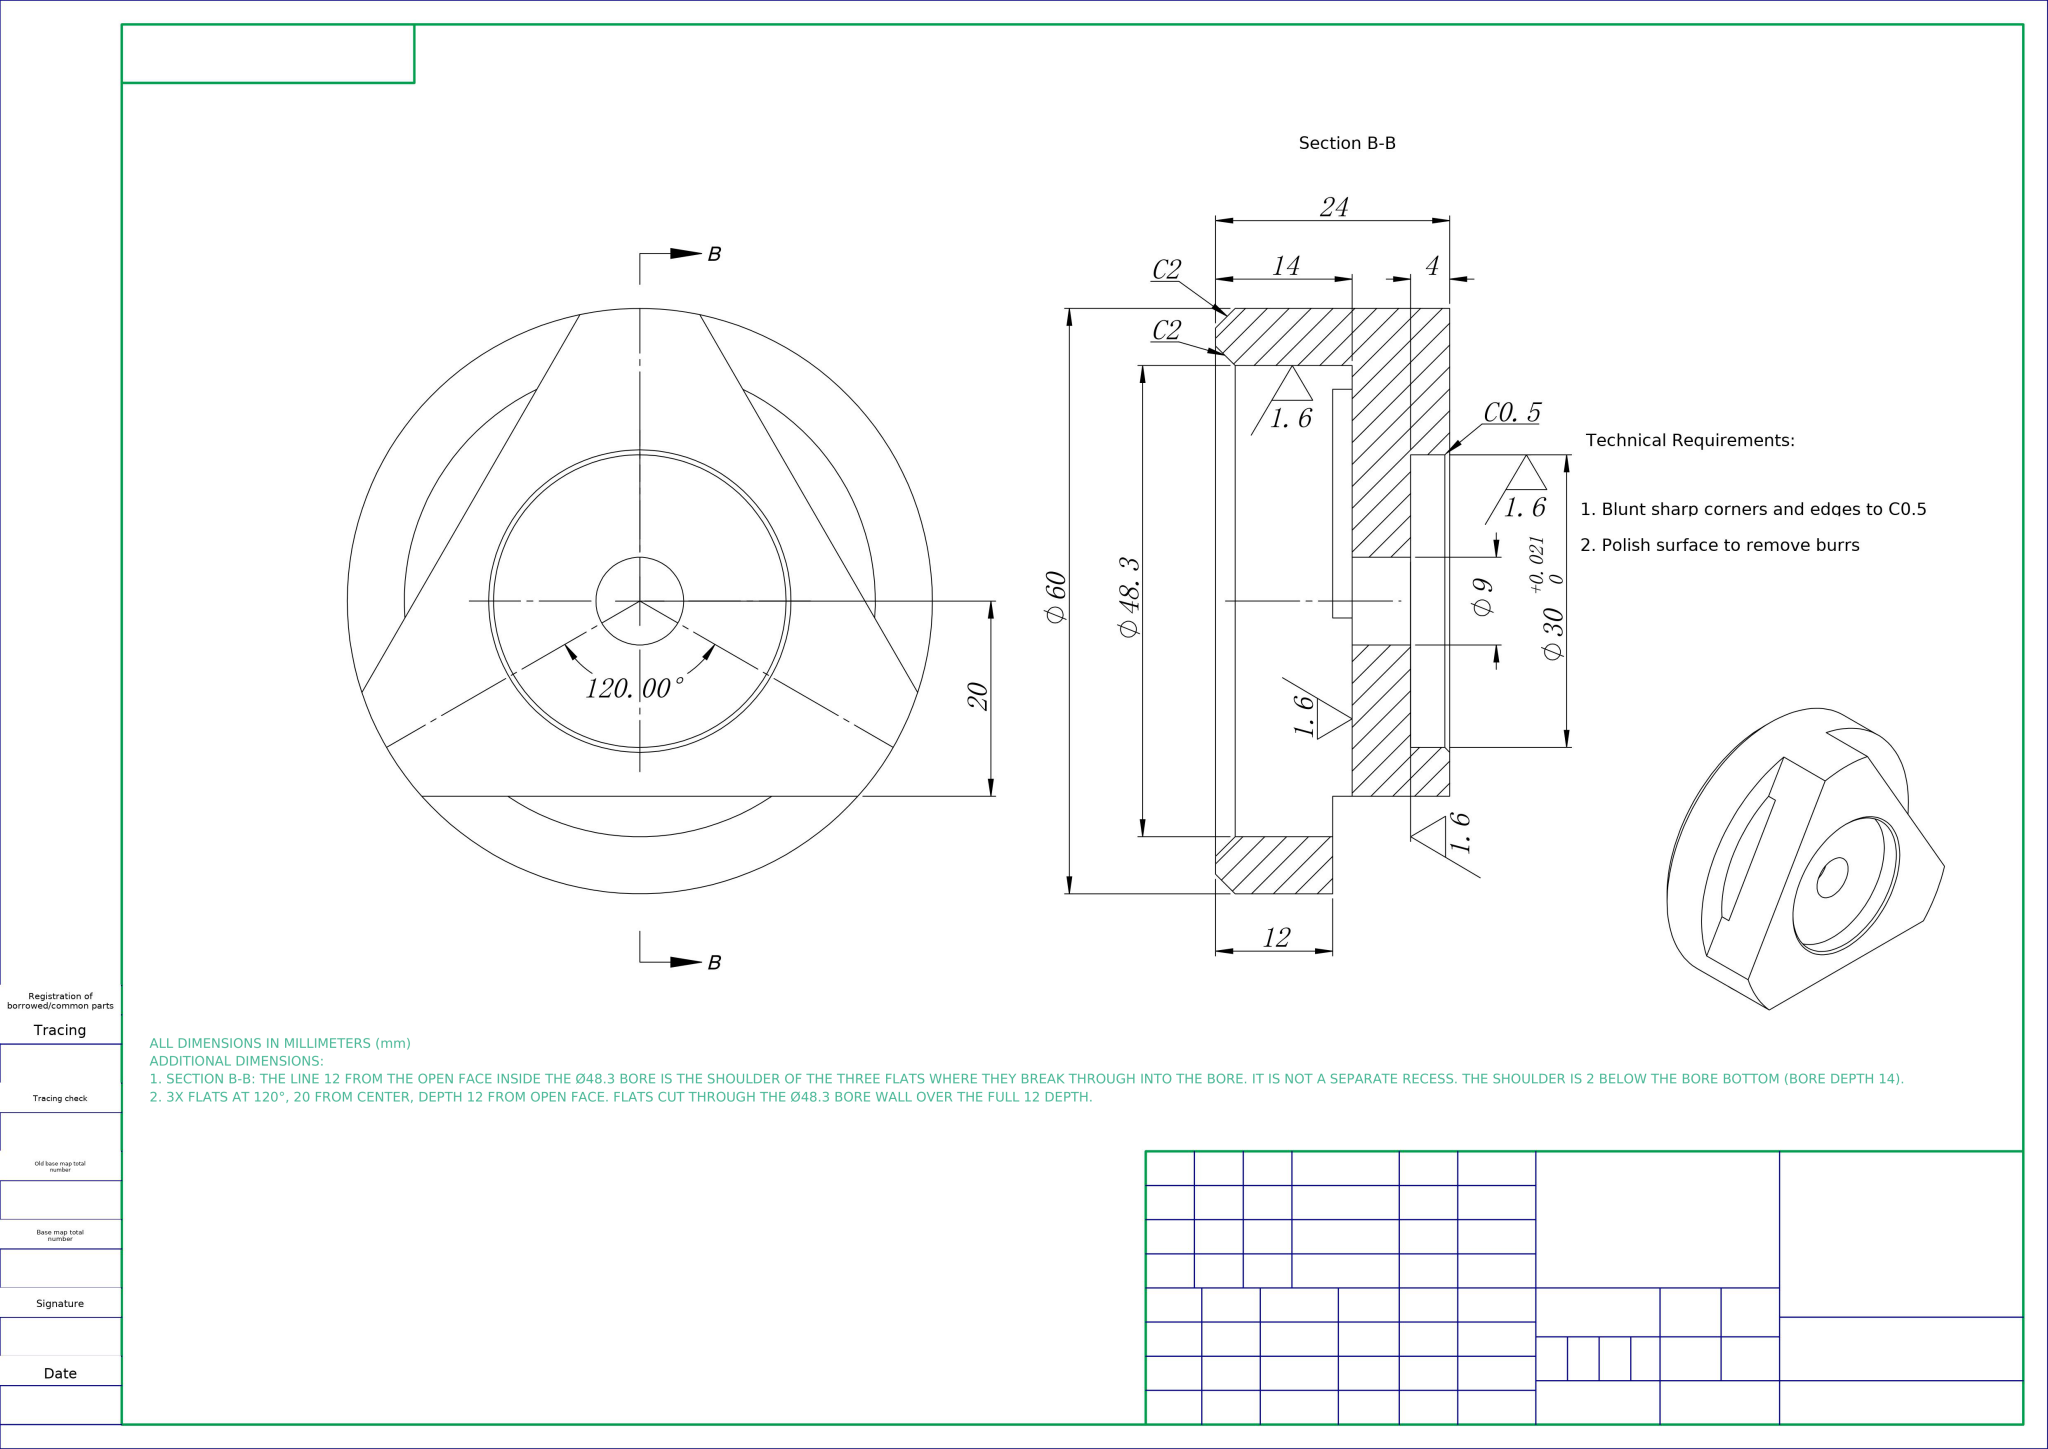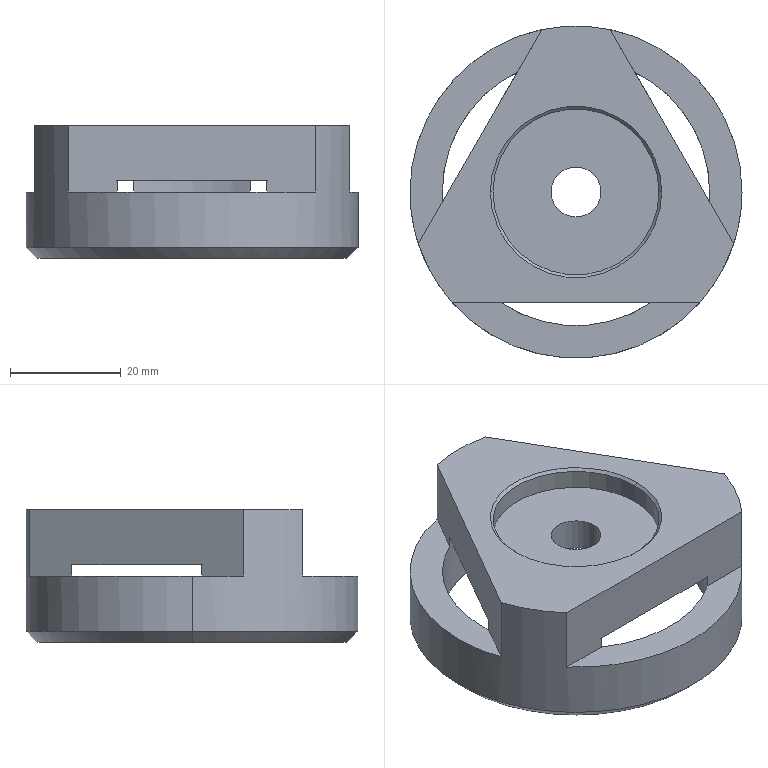Part | NX | mm | 1 solid | 24 faces | box 60 x 60 x 24 mm | volume 27612 mm3 | plane 10 | cylinder 8 | cone 6 | commonest cylinder face diameters 30 x2 48.3 x2 60 x2 9 x2
STEP:
#1=COLOUR_RGB('',0.,1.,1.);
#2=FILL_AREA_STYLE_COLOUR('',#1);
#3=FILL_AREA_STYLE('',(#2));
#4=SURFACE_STYLE_FILL_AREA(#3);
#5=SURFACE_SIDE_STYLE('',(#4));
#6=SURFACE_STYLE_USAGE(.BOTH.,#5);
#7=PRESENTATION_STYLE_ASSIGNMENT((#6));
#8=CARTESIAN_POINT('',(-15.,0.,23.5));
#9=VERTEX_POINT('',#8);
#10=CARTESIAN_POINT('',(15.,0.,23.5));
#11=VERTEX_POINT('',#10);
#12=CARTESIAN_POINT('',(0.,0.,23.5));
#13=DIRECTION('',(0.,0.,1.));
#14=DIRECTION('',(1.,0.,0.));
#15=AXIS2_PLACEMENT_3D('',#12,#13,#14);
#16=CIRCLE('',#15,15.);
#17=EDGE_CURVE('',#9,#11,#16,.T.);
#18=ORIENTED_EDGE('',*,*,#17,.F.);
#19=CARTESIAN_POINT('',(-15.5,0.,24.));
#20=VERTEX_POINT('',#19);
#21=CARTESIAN_POINT('',(-15.,0.,23.5));
#22=DIRECTION('',(-0.7071,0.,0.7071));
#23=VECTOR('',#22,1000.);
#24=LINE('',#21,#23);
#25=EDGE_CURVE('',#9,#20,#24,.T.);
#26=ORIENTED_EDGE('',*,*,#25,.T.);
#27=CARTESIAN_POINT('',(15.5,0.,24.));
#28=VERTEX_POINT('',#27);
#29=CARTESIAN_POINT('',(0.,0.,24.));
#30=DIRECTION('',(0.,0.,-1.));
#31=DIRECTION('',(1.,0.,0.));
#32=AXIS2_PLACEMENT_3D('',#29,#30,#31);
#33=CIRCLE('',#32,15.5);
#34=EDGE_CURVE('',#28,#20,#33,.T.);
#35=ORIENTED_EDGE('',*,*,#34,.F.);
#36=CARTESIAN_POINT('',(15.,0.,23.5));
#37=DIRECTION('',(0.7071,0.,0.7071));
#38=VECTOR('',#37,1000.);
#39=LINE('',#36,#38);
#40=EDGE_CURVE('',#11,#28,#39,.T.);
#41=ORIENTED_EDGE('',*,*,#40,.F.);
#42=EDGE_LOOP('',(#18,#26,#35,#41));
#43=FACE_OUTER_BOUND('',#42,.T.);
#44=CARTESIAN_POINT('',(0.,0.,23.5));
#45=DIRECTION('',(0.,0.,1.));
#46=DIRECTION('',(1.,0.,0.));
#47=AXIS2_PLACEMENT_3D('',#44,#45,#46);
#48=CONICAL_SURFACE('',#47,15.,0.7854);
#49=ADVANCED_FACE('',(#43),#48,.F.);
#50=CARTESIAN_POINT('',(-15.,0.,20.));
#51=VERTEX_POINT('',#50);
#52=CARTESIAN_POINT('',(15.,0.,20.));
#53=VERTEX_POINT('',#52);
#54=CARTESIAN_POINT('',(0.,0.,20.));
#55=DIRECTION('',(0.,0.,1.));
#56=DIRECTION('',(1.,0.,0.));
#57=AXIS2_PLACEMENT_3D('',#54,#55,#56);
#58=CIRCLE('',#57,15.);
#59=EDGE_CURVE('',#51,#53,#58,.T.);
#60=ORIENTED_EDGE('',*,*,#59,.F.);
#61=CARTESIAN_POINT('',(-15.,0.,20.));
#62=DIRECTION('',(0.,0.,1.));
#63=VECTOR('',#62,1000.);
#64=LINE('',#61,#63);
#65=EDGE_CURVE('',#51,#9,#64,.T.);
#66=ORIENTED_EDGE('',*,*,#65,.T.);
#67=ORIENTED_EDGE('',*,*,#17,.T.);
#68=CARTESIAN_POINT('',(15.,0.,20.));
#69=DIRECTION('',(0.,0.,1.));
#70=VECTOR('',#69,1000.);
#71=LINE('',#68,#70);
#72=EDGE_CURVE('',#53,#11,#71,.T.);
#73=ORIENTED_EDGE('',*,*,#72,.F.);
#74=EDGE_LOOP('',(#60,#66,#67,#73));
#75=FACE_OUTER_BOUND('',#74,.T.);
#76=CARTESIAN_POINT('',(0.,0.,20.));
#77=DIRECTION('',(0.,0.,1.));
#78=DIRECTION('',(1.,0.,0.));
#79=AXIS2_PLACEMENT_3D('',#76,#77,#78);
#80=CYLINDRICAL_SURFACE('',#79,15.);
#81=ADVANCED_FACE('',(#75),#80,.F.);
#82=CARTESIAN_POINT('',(24.15,0.,2.));
#83=VERTEX_POINT('',#82);
#84=CARTESIAN_POINT('',(-24.15,0.,2.));
#85=VERTEX_POINT('',#84);
#86=CARTESIAN_POINT('',(0.,0.,2.));
#87=DIRECTION('',(0.,0.,-1.));
#88=DIRECTION('',(1.,0.,0.));
#89=AXIS2_PLACEMENT_3D('',#86,#87,#88);
#90=CIRCLE('',#89,24.15);
#91=EDGE_CURVE('',#83,#85,#90,.T.);
#92=ORIENTED_EDGE('',*,*,#91,.F.);
#93=CARTESIAN_POINT('',(26.15,0.,0.));
#94=VERTEX_POINT('',#93);
#95=CARTESIAN_POINT('',(26.15,0.,0.));
#96=DIRECTION('',(0.7071,0.,-0.7071));
#97=VECTOR('',#96,1000.);
#98=LINE('',#95,#97);
#99=EDGE_CURVE('',#83,#94,#98,.T.);
#100=ORIENTED_EDGE('',*,*,#99,.T.);
#101=CARTESIAN_POINT('',(-26.15,0.,0.));
#102=VERTEX_POINT('',#101);
#103=CARTESIAN_POINT('',(0.,0.,0.));
#104=DIRECTION('',(0.,0.,1.));
#105=DIRECTION('',(1.,0.,0.));
#106=AXIS2_PLACEMENT_3D('',#103,#104,#105);
#107=CIRCLE('',#106,26.15);
#108=EDGE_CURVE('',#102,#94,#107,.T.);
#109=ORIENTED_EDGE('',*,*,#108,.F.);
#110=CARTESIAN_POINT('',(-26.15,0.,0.));
#111=DIRECTION('',(-0.7071,0.,-0.7071));
#112=VECTOR('',#111,1000.);
#113=LINE('',#110,#112);
#114=EDGE_CURVE('',#85,#102,#113,.T.);
#115=ORIENTED_EDGE('',*,*,#114,.F.);
#116=EDGE_LOOP('',(#92,#100,#109,#115));
#117=FACE_OUTER_BOUND('',#116,.T.);
#118=CARTESIAN_POINT('',(0.,0.,0.));
#119=DIRECTION('',(0.,0.,-1.));
#120=DIRECTION('',(-1.,0.,0.));
#121=AXIS2_PLACEMENT_3D('',#118,#119,#120);
#122=CONICAL_SURFACE('',#121,26.15,0.7854);
#123=ADVANCED_FACE('',(#117),#122,.F.);
#124=CARTESIAN_POINT('',(-28.,0.,0.));
#125=VERTEX_POINT('',#124);
#126=CARTESIAN_POINT('',(28.,0.,0.));
#127=VERTEX_POINT('',#126);
#128=CARTESIAN_POINT('',(0.,0.,0.));
#129=DIRECTION('',(0.,0.,-1.));
#130=DIRECTION('',(1.,0.,0.));
#131=AXIS2_PLACEMENT_3D('',#128,#129,#130);
#132=CIRCLE('',#131,28.);
#133=EDGE_CURVE('',#125,#127,#132,.T.);
#134=ORIENTED_EDGE('',*,*,#133,.F.);
#135=CARTESIAN_POINT('',(-30.,0.,2.));
#136=VERTEX_POINT('',#135);
#137=CARTESIAN_POINT('',(-30.,0.,2.));
#138=DIRECTION('',(-0.7071,0.,0.7071));
#139=VECTOR('',#138,1000.);
#140=LINE('',#137,#139);
#141=EDGE_CURVE('',#125,#136,#140,.T.);
#142=ORIENTED_EDGE('',*,*,#141,.T.);
#143=CARTESIAN_POINT('',(30.,0.,2.));
#144=VERTEX_POINT('',#143);
#145=CARTESIAN_POINT('',(0.,0.,2.));
#146=DIRECTION('',(0.,0.,1.));
#147=DIRECTION('',(1.,0.,0.));
#148=AXIS2_PLACEMENT_3D('',#145,#146,#147);
#149=CIRCLE('',#148,30.);
#150=EDGE_CURVE('',#144,#136,#149,.T.);
#151=ORIENTED_EDGE('',*,*,#150,.F.);
#152=CARTESIAN_POINT('',(30.,0.,2.));
#153=DIRECTION('',(0.7071,0.,0.7071));
#154=VECTOR('',#153,1000.);
#155=LINE('',#152,#154);
#156=EDGE_CURVE('',#127,#144,#155,.T.);
#157=ORIENTED_EDGE('',*,*,#156,.F.);
#158=EDGE_LOOP('',(#134,#142,#151,#157));
#159=FACE_OUTER_BOUND('',#158,.T.);
#160=CARTESIAN_POINT('',(0.,0.,2.));
#161=DIRECTION('',(0.,0.,1.));
#162=DIRECTION('',(1.,0.,0.));
#163=AXIS2_PLACEMENT_3D('',#160,#161,#162);
#164=CONICAL_SURFACE('',#163,30.,0.7854);
#165=ADVANCED_FACE('',(#159),#164,.T.);
#166=CARTESIAN_POINT('',(24.088,-1.722,12.));
#167=VERTEX_POINT('',#166);
#168=CARTESIAN_POINT('',(24.15,0.,12.));
#169=VERTEX_POINT('',#168);
#170=CARTESIAN_POINT('',(0.,0.,12.));
#171=DIRECTION('',(0.,0.,1.));
#172=DIRECTION('',(1.,0.,0.));
#173=AXIS2_PLACEMENT_3D('',#170,#171,#172);
#174=CIRCLE('',#173,24.15);
#175=EDGE_CURVE('',#167,#169,#174,.T.);
#176=ORIENTED_EDGE('',*,*,#175,.T.);
#177=CARTESIAN_POINT('',(24.15,0.,14.));
#178=DIRECTION('',(0.,0.,-1.));
#179=VECTOR('',#178,1000.);
#180=LINE('',#177,#179);
#181=EDGE_CURVE('',#169,#83,#180,.T.);
#182=ORIENTED_EDGE('',*,*,#181,.T.);
#183=ORIENTED_EDGE('',*,*,#91,.T.);
#184=CARTESIAN_POINT('',(-24.15,0.,12.));
#185=VERTEX_POINT('',#184);
#186=CARTESIAN_POINT('',(-24.15,0.,14.));
#187=DIRECTION('',(0.,0.,-1.));
#188=VECTOR('',#187,1000.);
#189=LINE('',#186,#188);
#190=EDGE_CURVE('',#185,#85,#189,.T.);
#191=ORIENTED_EDGE('',*,*,#190,.F.);
#192=CARTESIAN_POINT('',(-24.088,-1.722,12.));
#193=VERTEX_POINT('',#192);
#194=CARTESIAN_POINT('',(0.,0.,12.));
#195=DIRECTION('',(0.,0.,1.));
#196=DIRECTION('',(1.,0.,0.));
#197=AXIS2_PLACEMENT_3D('',#194,#195,#196);
#198=CIRCLE('',#197,24.15);
#199=EDGE_CURVE('',#185,#193,#198,.T.);
#200=ORIENTED_EDGE('',*,*,#199,.T.);
#201=CARTESIAN_POINT('',(-24.088,-1.722,14.));
#202=VERTEX_POINT('',#201);
#203=CARTESIAN_POINT('',(-24.088,-1.722,14.));
#204=DIRECTION('',(0.,0.,-1.));
#205=VECTOR('',#204,1000.);
#206=LINE('',#203,#205);
#207=EDGE_CURVE('',#202,#193,#206,.T.);
#208=ORIENTED_EDGE('',*,*,#207,.F.);
#209=CARTESIAN_POINT('',(-13.536,-20.,14.));
#210=VERTEX_POINT('',#209);
#211=CARTESIAN_POINT('',(0.,0.,14.));
#212=DIRECTION('',(0.,0.,1.));
#213=DIRECTION('',(1.,0.,0.));
#214=AXIS2_PLACEMENT_3D('',#211,#212,#213);
#215=CIRCLE('',#214,24.15);
#216=EDGE_CURVE('',#202,#210,#215,.T.);
#217=ORIENTED_EDGE('',*,*,#216,.T.);
#218=CARTESIAN_POINT('',(-13.536,-20.,12.));
#219=VERTEX_POINT('',#218);
#220=CARTESIAN_POINT('',(-13.536,-20.,14.));
#221=DIRECTION('',(0.,0.,1.));
#222=VECTOR('',#221,1000.);
#223=LINE('',#220,#222);
#224=EDGE_CURVE('',#219,#210,#223,.T.);
#225=ORIENTED_EDGE('',*,*,#224,.F.);
#226=CARTESIAN_POINT('',(13.536,-20.,12.));
#227=VERTEX_POINT('',#226);
#228=CARTESIAN_POINT('',(0.,0.,12.));
#229=DIRECTION('',(0.,0.,1.));
#230=DIRECTION('',(1.,0.,0.));
#231=AXIS2_PLACEMENT_3D('',#228,#229,#230);
#232=CIRCLE('',#231,24.15);
#233=EDGE_CURVE('',#219,#227,#232,.T.);
#234=ORIENTED_EDGE('',*,*,#233,.T.);
#235=CARTESIAN_POINT('',(13.536,-20.,14.));
#236=VERTEX_POINT('',#235);
#237=CARTESIAN_POINT('',(13.536,-20.,14.));
#238=DIRECTION('',(0.,0.,-1.));
#239=VECTOR('',#238,1000.);
#240=LINE('',#237,#239);
#241=EDGE_CURVE('',#236,#227,#240,.T.);
#242=ORIENTED_EDGE('',*,*,#241,.F.);
#243=CARTESIAN_POINT('',(24.088,-1.722,14.));
#244=VERTEX_POINT('',#243);
#245=CARTESIAN_POINT('',(0.,0.,14.));
#246=DIRECTION('',(0.,0.,1.));
#247=DIRECTION('',(1.,0.,0.));
#248=AXIS2_PLACEMENT_3D('',#245,#246,#247);
#249=CIRCLE('',#248,24.15);
#250=EDGE_CURVE('',#236,#244,#249,.T.);
#251=ORIENTED_EDGE('',*,*,#250,.T.);
#252=CARTESIAN_POINT('',(24.088,-1.722,14.));
#253=DIRECTION('',(0.,0.,1.));
#254=VECTOR('',#253,1000.);
#255=LINE('',#252,#254);
#256=EDGE_CURVE('',#167,#244,#255,.T.);
#257=ORIENTED_EDGE('',*,*,#256,.F.);
#258=EDGE_LOOP('',(#176,#182,#183,#191,#200,#208,#217,#225,#234,#242,#251,#257));
#259=FACE_OUTER_BOUND('',#258,.T.);
#260=CARTESIAN_POINT('',(0.,0.,14.));
#261=DIRECTION('',(0.,0.,-1.));
#262=DIRECTION('',(-1.,0.,0.));
#263=AXIS2_PLACEMENT_3D('',#260,#261,#262);
#264=CYLINDRICAL_SURFACE('',#263,24.15);
#265=ADVANCED_FACE('',(#259),#264,.F.);
#266=CARTESIAN_POINT('',(30.,0.,12.));
#267=VERTEX_POINT('',#266);
#268=CARTESIAN_POINT('',(6.14,29.365,12.));
#269=VERTEX_POINT('',#268);
#270=CARTESIAN_POINT('',(0.,0.,12.));
#271=DIRECTION('',(0.,0.,1.));
#272=DIRECTION('',(-0.5,-0.866,0.));
#273=AXIS2_PLACEMENT_3D('',#270,#271,#272);
#274=CIRCLE('',#273,30.);
#275=EDGE_CURVE('',#267,#269,#274,.T.);
#276=ORIENTED_EDGE('',*,*,#275,.F.);
#277=CARTESIAN_POINT('',(30.,0.,14.));
#278=DIRECTION('',(0.,0.,-1.));
#279=VECTOR('',#278,1000.);
#280=LINE('',#277,#279);
#281=EDGE_CURVE('',#267,#144,#280,.T.);
#282=ORIENTED_EDGE('',*,*,#281,.T.);
#283=ORIENTED_EDGE('',*,*,#150,.T.);
#284=CARTESIAN_POINT('',(-30.,0.,12.));
#285=VERTEX_POINT('',#284);
#286=CARTESIAN_POINT('',(-30.,0.,14.));
#287=DIRECTION('',(0.,0.,-1.));
#288=VECTOR('',#287,1000.);
#289=LINE('',#286,#288);
#290=EDGE_CURVE('',#285,#136,#289,.T.);
#291=ORIENTED_EDGE('',*,*,#290,.F.);
#292=CARTESIAN_POINT('',(-6.14,29.365,12.));
#293=VERTEX_POINT('',#292);
#294=CARTESIAN_POINT('',(0.,0.,12.));
#295=DIRECTION('',(0.,0.,1.));
#296=DIRECTION('',(1.,0.,0.));
#297=AXIS2_PLACEMENT_3D('',#294,#295,#296);
#298=CIRCLE('',#297,30.);
#299=EDGE_CURVE('',#293,#285,#298,.T.);
#300=ORIENTED_EDGE('',*,*,#299,.F.);
#301=CARTESIAN_POINT('',(-6.14,29.365,24.));
#302=VERTEX_POINT('',#301);
#303=CARTESIAN_POINT('',(-6.14,29.365,12.));
#304=DIRECTION('',(0.,0.,1.));
#305=VECTOR('',#304,1000.);
#306=LINE('',#303,#305);
#307=EDGE_CURVE('',#293,#302,#306,.T.);
#308=ORIENTED_EDGE('',*,*,#307,.T.);
#309=CARTESIAN_POINT('',(6.14,29.365,24.));
#310=VERTEX_POINT('',#309);
#311=CARTESIAN_POINT('',(0.,0.,24.));
#312=DIRECTION('',(0.,0.,1.));
#313=DIRECTION('',(1.,0.,0.));
#314=AXIS2_PLACEMENT_3D('',#311,#312,#313);
#315=CIRCLE('',#314,30.);
#316=EDGE_CURVE('',#310,#302,#315,.T.);
#317=ORIENTED_EDGE('',*,*,#316,.F.);
#318=CARTESIAN_POINT('',(6.14,29.365,12.));
#319=DIRECTION('',(0.,0.,1.));
#320=VECTOR('',#319,1000.);
#321=LINE('',#318,#320);
#322=EDGE_CURVE('',#269,#310,#321,.T.);
#323=ORIENTED_EDGE('',*,*,#322,.F.);
#324=EDGE_LOOP('',(#276,#282,#283,#291,#300,#308,#317,#323));
#325=FACE_OUTER_BOUND('',#324,.T.);
#326=CARTESIAN_POINT('',(0.,0.,14.));
#327=DIRECTION('',(0.,0.,-1.));
#328=DIRECTION('',(-1.,0.,0.));
#329=AXIS2_PLACEMENT_3D('',#326,#327,#328);
#330=CYLINDRICAL_SURFACE('',#329,30.);
#331=ADVANCED_FACE('',(#325),#330,.T.);
#332=CARTESIAN_POINT('',(4.5,0.,20.));
#333=VERTEX_POINT('',#332);
#334=CARTESIAN_POINT('',(-4.5,0.,20.));
#335=VERTEX_POINT('',#334);
#336=CARTESIAN_POINT('',(0.,0.,20.));
#337=DIRECTION('',(0.,0.,-1.));
#338=DIRECTION('',(1.,0.,0.));
#339=AXIS2_PLACEMENT_3D('',#336,#337,#338);
#340=CIRCLE('',#339,4.5);
#341=EDGE_CURVE('',#333,#335,#340,.T.);
#342=ORIENTED_EDGE('',*,*,#341,.F.);
#343=CARTESIAN_POINT('',(4.5,0.,14.));
#344=VERTEX_POINT('',#343);
#345=CARTESIAN_POINT('',(4.5,0.,14.));
#346=DIRECTION('',(0.,0.,-1.));
#347=VECTOR('',#346,1000.);
#348=LINE('',#345,#347);
#349=EDGE_CURVE('',#333,#344,#348,.T.);
#350=ORIENTED_EDGE('',*,*,#349,.T.);
#351=CARTESIAN_POINT('',(-4.5,0.,14.));
#352=VERTEX_POINT('',#351);
#353=CARTESIAN_POINT('',(0.,0.,14.));
#354=DIRECTION('',(0.,0.,-1.));
#355=DIRECTION('',(-1.,0.,0.));
#356=AXIS2_PLACEMENT_3D('',#353,#354,#355);
#357=CIRCLE('',#356,4.5);
#358=EDGE_CURVE('',#344,#352,#357,.T.);
#359=ORIENTED_EDGE('',*,*,#358,.T.);
#360=CARTESIAN_POINT('',(-4.5,0.,14.));
#361=DIRECTION('',(0.,0.,-1.));
#362=VECTOR('',#361,1000.);
#363=LINE('',#360,#362);
#364=EDGE_CURVE('',#335,#352,#363,.T.);
#365=ORIENTED_EDGE('',*,*,#364,.F.);
#366=EDGE_LOOP('',(#342,#350,#359,#365));
#367=FACE_OUTER_BOUND('',#366,.T.);
#368=CARTESIAN_POINT('',(0.,0.,14.));
#369=DIRECTION('',(0.,0.,-1.));
#370=DIRECTION('',(-1.,0.,0.));
#371=AXIS2_PLACEMENT_3D('',#368,#369,#370);
#372=CYLINDRICAL_SURFACE('',#371,4.5);
#373=ADVANCED_FACE('',(#367),#372,.F.);
#374=ORIENTED_EDGE('',*,*,#349,.F.);
#375=CARTESIAN_POINT('',(0.,0.,20.));
#376=DIRECTION('',(0.,0.,-1.));
#377=DIRECTION('',(1.,0.,0.));
#378=AXIS2_PLACEMENT_3D('',#375,#376,#377);
#379=CIRCLE('',#378,4.5);
#380=EDGE_CURVE('',#335,#333,#379,.T.);
#381=ORIENTED_EDGE('',*,*,#380,.F.);
#382=ORIENTED_EDGE('',*,*,#364,.T.);
#383=CARTESIAN_POINT('',(0.,0.,14.));
#384=DIRECTION('',(0.,0.,-1.));
#385=DIRECTION('',(-1.,0.,0.));
#386=AXIS2_PLACEMENT_3D('',#383,#384,#385);
#387=CIRCLE('',#386,4.5);
#388=EDGE_CURVE('',#352,#344,#387,.T.);
#389=ORIENTED_EDGE('',*,*,#388,.T.);
#390=EDGE_LOOP('',(#374,#381,#382,#389));
#391=FACE_OUTER_BOUND('',#390,.T.);
#392=CARTESIAN_POINT('',(0.,0.,14.));
#393=DIRECTION('',(0.,0.,-1.));
#394=DIRECTION('',(-1.,0.,0.));
#395=AXIS2_PLACEMENT_3D('',#392,#393,#394);
#396=CYLINDRICAL_SURFACE('',#395,4.5);
#397=ADVANCED_FACE('',(#391),#396,.F.);
#398=CARTESIAN_POINT('',(0.,0.,0.));
#399=DIRECTION('',(0.,0.,-1.));
#400=DIRECTION('',(1.,0.,0.));
#401=AXIS2_PLACEMENT_3D('',#398,#399,#400);
#402=CIRCLE('',#401,28.);
#403=EDGE_CURVE('',#127,#125,#402,.T.);
#404=ORIENTED_EDGE('',*,*,#403,.T.);
#405=ORIENTED_EDGE('',*,*,#133,.T.);
#406=EDGE_LOOP('',(#404,#405));
#407=FACE_OUTER_BOUND('',#406,.T.);
#408=ORIENTED_EDGE('',*,*,#108,.T.);
#409=CARTESIAN_POINT('',(0.,0.,0.));
#410=DIRECTION('',(0.,0.,1.));
#411=DIRECTION('',(1.,0.,0.));
#412=AXIS2_PLACEMENT_3D('',#409,#410,#411);
#413=CIRCLE('',#412,26.15);
#414=EDGE_CURVE('',#94,#102,#413,.T.);
#415=ORIENTED_EDGE('',*,*,#414,.T.);
#416=EDGE_LOOP('',(#408,#415));
#417=FACE_BOUND('',#416,.T.);
#418=CARTESIAN_POINT('',(0.,0.,0.));
#419=DIRECTION('',(0.,0.,1.));
#420=DIRECTION('',(1.,0.,0.));
#421=AXIS2_PLACEMENT_3D('',#418,#419,#420);
#422=PLANE('',#421);
#423=ADVANCED_FACE('',(#407,#417),#422,.F.);
#424=ORIENTED_EDGE('',*,*,#281,.F.);
#425=CARTESIAN_POINT('',(28.501,-9.365,12.));
#426=VERTEX_POINT('',#425);
#427=CARTESIAN_POINT('',(0.,0.,12.));
#428=DIRECTION('',(0.,0.,1.));
#429=DIRECTION('',(-0.5,-0.866,0.));
#430=AXIS2_PLACEMENT_3D('',#427,#428,#429);
#431=CIRCLE('',#430,30.);
#432=EDGE_CURVE('',#426,#267,#431,.T.);
#433=ORIENTED_EDGE('',*,*,#432,.F.);
#434=CARTESIAN_POINT('',(28.501,-9.365,24.));
#435=VERTEX_POINT('',#434);
#436=CARTESIAN_POINT('',(28.501,-9.365,12.));
#437=DIRECTION('',(0.,0.,1.));
#438=VECTOR('',#437,1000.);
#439=LINE('',#436,#438);
#440=EDGE_CURVE('',#426,#435,#439,.T.);
#441=ORIENTED_EDGE('',*,*,#440,.T.);
#442=CARTESIAN_POINT('',(22.361,-20.,24.));
#443=VERTEX_POINT('',#442);
#444=CARTESIAN_POINT('',(0.,0.,24.));
#445=DIRECTION('',(0.,0.,1.));
#446=DIRECTION('',(1.,0.,0.));
#447=AXIS2_PLACEMENT_3D('',#444,#445,#446);
#448=CIRCLE('',#447,30.);
#449=EDGE_CURVE('',#443,#435,#448,.T.);
#450=ORIENTED_EDGE('',*,*,#449,.F.);
#451=CARTESIAN_POINT('',(22.361,-20.,12.));
#452=VERTEX_POINT('',#451);
#453=CARTESIAN_POINT('',(22.361,-20.,12.));
#454=DIRECTION('',(0.,0.,1.));
#455=VECTOR('',#454,1000.);
#456=LINE('',#453,#455);
#457=EDGE_CURVE('',#452,#443,#456,.T.);
#458=ORIENTED_EDGE('',*,*,#457,.F.);
#459=CARTESIAN_POINT('',(-22.361,-20.,12.));
#460=VERTEX_POINT('',#459);
#461=CARTESIAN_POINT('',(0.,0.,12.));
#462=DIRECTION('',(0.,0.,1.));
#463=DIRECTION('',(-0.5,0.866,0.));
#464=AXIS2_PLACEMENT_3D('',#461,#462,#463);
#465=CIRCLE('',#464,30.);
#466=EDGE_CURVE('',#460,#452,#465,.T.);
#467=ORIENTED_EDGE('',*,*,#466,.F.);
#468=CARTESIAN_POINT('',(-22.361,-20.,24.));
#469=VERTEX_POINT('',#468);
#470=CARTESIAN_POINT('',(-22.361,-20.,12.));
#471=DIRECTION('',(0.,0.,1.));
#472=VECTOR('',#471,1000.);
#473=LINE('',#470,#472);
#474=EDGE_CURVE('',#460,#469,#473,.T.);
#475=ORIENTED_EDGE('',*,*,#474,.T.);
#476=CARTESIAN_POINT('',(-28.501,-9.365,24.));
#477=VERTEX_POINT('',#476);
#478=CARTESIAN_POINT('',(0.,0.,24.));
#479=DIRECTION('',(0.,0.,1.));
#480=DIRECTION('',(1.,0.,0.));
#481=AXIS2_PLACEMENT_3D('',#478,#479,#480);
#482=CIRCLE('',#481,30.);
#483=EDGE_CURVE('',#477,#469,#482,.T.);
#484=ORIENTED_EDGE('',*,*,#483,.F.);
#485=CARTESIAN_POINT('',(-28.501,-9.365,12.));
#486=VERTEX_POINT('',#485);
#487=CARTESIAN_POINT('',(-28.501,-9.365,12.));
#488=DIRECTION('',(0.,0.,1.));
#489=VECTOR('',#488,1000.);
#490=LINE('',#487,#489);
#491=EDGE_CURVE('',#486,#477,#490,.T.);
#492=ORIENTED_EDGE('',*,*,#491,.F.);
#493=CARTESIAN_POINT('',(0.,0.,12.));
#494=DIRECTION('',(0.,0.,1.));
#495=DIRECTION('',(1.,0.,0.));
#496=AXIS2_PLACEMENT_3D('',#493,#494,#495);
#497=CIRCLE('',#496,30.);
#498=EDGE_CURVE('',#285,#486,#497,.T.);
#499=ORIENTED_EDGE('',*,*,#498,.F.);
#500=ORIENTED_EDGE('',*,*,#290,.T.);
#501=CARTESIAN_POINT('',(0.,0.,2.));
#502=DIRECTION('',(0.,0.,1.));
#503=DIRECTION('',(1.,0.,0.));
#504=AXIS2_PLACEMENT_3D('',#501,#502,#503);
#505=CIRCLE('',#504,30.);
#506=EDGE_CURVE('',#136,#144,#505,.T.);
#507=ORIENTED_EDGE('',*,*,#506,.T.);
#508=EDGE_LOOP('',(#424,#433,#441,#450,#458,#467,#475,#484,#492,#499,#500,#507));
#509=FACE_OUTER_BOUND('',#508,.T.);
#510=CARTESIAN_POINT('',(0.,0.,14.));
#511=DIRECTION('',(0.,0.,-1.));
#512=DIRECTION('',(-1.,0.,0.));
#513=AXIS2_PLACEMENT_3D('',#510,#511,#512);
#514=CYLINDRICAL_SURFACE('',#513,30.);
#515=ADVANCED_FACE('',(#509),#514,.T.);
#516=ORIENTED_EDGE('',*,*,#181,.F.);
#517=CARTESIAN_POINT('',(10.553,21.722,12.));
#518=VERTEX_POINT('',#517);
#519=CARTESIAN_POINT('',(0.,0.,12.));
#520=DIRECTION('',(0.,0.,1.));
#521=DIRECTION('',(1.,0.,0.));
#522=AXIS2_PLACEMENT_3D('',#519,#520,#521);
#523=CIRCLE('',#522,24.15);
#524=EDGE_CURVE('',#169,#518,#523,.T.);
#525=ORIENTED_EDGE('',*,*,#524,.T.);
#526=CARTESIAN_POINT('',(10.553,21.722,14.));
#527=VERTEX_POINT('',#526);
#528=CARTESIAN_POINT('',(10.553,21.722,14.));
#529=DIRECTION('',(0.,0.,-1.));
#530=VECTOR('',#529,1000.);
#531=LINE('',#528,#530);
#532=EDGE_CURVE('',#527,#518,#531,.T.);
#533=ORIENTED_EDGE('',*,*,#532,.F.);
#534=CARTESIAN_POINT('',(-10.553,21.722,14.));
#535=VERTEX_POINT('',#534);
#536=CARTESIAN_POINT('',(0.,0.,14.));
#537=DIRECTION('',(0.,0.,1.));
#538=DIRECTION('',(1.,0.,0.));
#539=AXIS2_PLACEMENT_3D('',#536,#537,#538);
#540=CIRCLE('',#539,24.15);
#541=EDGE_CURVE('',#527,#535,#540,.T.);
#542=ORIENTED_EDGE('',*,*,#541,.T.);
#543=CARTESIAN_POINT('',(-10.553,21.722,12.));
#544=VERTEX_POINT('',#543);
#545=CARTESIAN_POINT('',(-10.553,21.722,14.));
#546=DIRECTION('',(0.,0.,1.));
#547=VECTOR('',#546,1000.);
#548=LINE('',#545,#547);
#549=EDGE_CURVE('',#544,#535,#548,.T.);
#550=ORIENTED_EDGE('',*,*,#549,.F.);
#551=CARTESIAN_POINT('',(0.,0.,12.));
#552=DIRECTION('',(0.,0.,1.));
#553=DIRECTION('',(1.,0.,0.));
#554=AXIS2_PLACEMENT_3D('',#551,#552,#553);
#555=CIRCLE('',#554,24.15);
#556=EDGE_CURVE('',#544,#185,#555,.T.);
#557=ORIENTED_EDGE('',*,*,#556,.T.);
#558=ORIENTED_EDGE('',*,*,#190,.T.);
#559=CARTESIAN_POINT('',(0.,0.,2.));
#560=DIRECTION('',(0.,0.,-1.));
#561=DIRECTION('',(1.,0.,0.));
#562=AXIS2_PLACEMENT_3D('',#559,#560,#561);
#563=CIRCLE('',#562,24.15);
#564=EDGE_CURVE('',#85,#83,#563,.T.);
#565=ORIENTED_EDGE('',*,*,#564,.T.);
#566=EDGE_LOOP('',(#516,#525,#533,#542,#550,#557,#558,#565));
#567=FACE_OUTER_BOUND('',#566,.T.);
#568=CARTESIAN_POINT('',(0.,0.,14.));
#569=DIRECTION('',(0.,0.,-1.));
#570=DIRECTION('',(-1.,0.,0.));
#571=AXIS2_PLACEMENT_3D('',#568,#569,#570);
#572=CYLINDRICAL_SURFACE('',#571,24.15);
#573=ADVANCED_FACE('',(#567),#572,.F.);
#574=ORIENTED_EDGE('',*,*,#141,.F.);
#575=ORIENTED_EDGE('',*,*,#403,.F.);
#576=ORIENTED_EDGE('',*,*,#156,.T.);
#577=ORIENTED_EDGE('',*,*,#506,.F.);
#578=EDGE_LOOP('',(#574,#575,#576,#577));
#579=FACE_OUTER_BOUND('',#578,.T.);
#580=CARTESIAN_POINT('',(0.,0.,2.));
#581=DIRECTION('',(0.,0.,1.));
#582=DIRECTION('',(1.,0.,0.));
#583=AXIS2_PLACEMENT_3D('',#580,#581,#582);
#584=CONICAL_SURFACE('',#583,30.,0.7854);
#585=ADVANCED_FACE('',(#579),#584,.T.);
#586=ORIENTED_EDGE('',*,*,#99,.F.);
#587=ORIENTED_EDGE('',*,*,#564,.F.);
#588=ORIENTED_EDGE('',*,*,#114,.T.);
#589=ORIENTED_EDGE('',*,*,#414,.F.);
#590=EDGE_LOOP('',(#586,#587,#588,#589));
#591=FACE_OUTER_BOUND('',#590,.T.);
#592=CARTESIAN_POINT('',(0.,0.,0.));
#593=DIRECTION('',(0.,0.,-1.));
#594=DIRECTION('',(-1.,0.,0.));
#595=AXIS2_PLACEMENT_3D('',#592,#593,#594);
#596=CONICAL_SURFACE('',#595,26.15,0.7854);
#597=ADVANCED_FACE('',(#591),#596,.F.);
#598=ORIENTED_EDGE('',*,*,#388,.F.);
#599=ORIENTED_EDGE('',*,*,#358,.F.);
#600=EDGE_LOOP('',(#598,#599));
#601=FACE_BOUND('',#600,.T.);
#602=ORIENTED_EDGE('',*,*,#250,.F.);
#603=CARTESIAN_POINT('',(-0.,-20.,14.));
#604=DIRECTION('',(-1.,0.,0.));
#605=VECTOR('',#604,1000.);
#606=LINE('',#603,#605);
#607=EDGE_CURVE('',#236,#210,#606,.T.);
#608=ORIENTED_EDGE('',*,*,#607,.T.);
#609=ORIENTED_EDGE('',*,*,#216,.F.);
#610=CARTESIAN_POINT('',(-17.321,10.,14.));
#611=DIRECTION('',(0.5,0.866,0.));
#612=VECTOR('',#611,1000.);
#613=LINE('',#610,#612);
#614=EDGE_CURVE('',#202,#535,#613,.T.);
#615=ORIENTED_EDGE('',*,*,#614,.T.);
#616=ORIENTED_EDGE('',*,*,#541,.F.);
#617=CARTESIAN_POINT('',(17.321,10.,14.));
#618=DIRECTION('',(0.5,-0.866,0.));
#619=VECTOR('',#618,1000.);
#620=LINE('',#617,#619);
#621=EDGE_CURVE('',#527,#244,#620,.T.);
#622=ORIENTED_EDGE('',*,*,#621,.T.);
#623=EDGE_LOOP('',(#602,#608,#609,#615,#616,#622));
#624=FACE_OUTER_BOUND('',#623,.T.);
#625=CARTESIAN_POINT('',(0.,0.,14.));
#626=DIRECTION('',(0.,0.,1.));
#627=DIRECTION('',(1.,0.,0.));
#628=AXIS2_PLACEMENT_3D('',#625,#626,#627);
#629=PLANE('',#628);
#630=ADVANCED_FACE('',(#601,#624),#629,.F.);
#631=ORIENTED_EDGE('',*,*,#34,.T.);
#632=CARTESIAN_POINT('',(0.,0.,24.));
#633=DIRECTION('',(0.,0.,-1.));
#634=DIRECTION('',(1.,0.,0.));
#635=AXIS2_PLACEMENT_3D('',#632,#633,#634);
#636=CIRCLE('',#635,15.5);
#637=EDGE_CURVE('',#20,#28,#636,.T.);
#638=ORIENTED_EDGE('',*,*,#637,.T.);
#639=EDGE_LOOP('',(#631,#638));
#640=FACE_BOUND('',#639,.T.);
#641=CARTESIAN_POINT('',(-22.361,-20.,24.));
#642=DIRECTION('',(-1.,0.,0.));
#643=VECTOR('',#642,1000.);
#644=LINE('',#641,#643);
#645=EDGE_CURVE('',#443,#469,#644,.T.);
#646=ORIENTED_EDGE('',*,*,#645,.F.);
#647=ORIENTED_EDGE('',*,*,#449,.T.);
#648=CARTESIAN_POINT('',(28.501,-9.365,24.));
#649=DIRECTION('',(0.5,-0.866,0.));
#650=VECTOR('',#649,1000.);
#651=LINE('',#648,#650);
#652=EDGE_CURVE('',#310,#435,#651,.T.);
#653=ORIENTED_EDGE('',*,*,#652,.F.);
#654=ORIENTED_EDGE('',*,*,#316,.T.);
#655=CARTESIAN_POINT('',(-6.14,29.365,24.));
#656=DIRECTION('',(0.5,0.866,0.));
#657=VECTOR('',#656,1000.);
#658=LINE('',#655,#657);
#659=EDGE_CURVE('',#477,#302,#658,.T.);
#660=ORIENTED_EDGE('',*,*,#659,.F.);
#661=ORIENTED_EDGE('',*,*,#483,.T.);
#662=EDGE_LOOP('',(#646,#647,#653,#654,#660,#661));
#663=FACE_OUTER_BOUND('',#662,.T.);
#664=CARTESIAN_POINT('',(0.,0.,24.));
#665=DIRECTION('',(0.,0.,1.));
#666=DIRECTION('',(1.,0.,0.));
#667=AXIS2_PLACEMENT_3D('',#664,#665,#666);
#668=PLANE('',#667);
#669=ADVANCED_FACE('',(#640,#663),#668,.T.);
#670=ORIENTED_EDGE('',*,*,#207,.T.);
#671=CARTESIAN_POINT('',(-6.14,29.365,12.));
#672=DIRECTION('',(0.5,0.866,0.));
#673=VECTOR('',#672,1000.);
#674=LINE('',#671,#673);
#675=EDGE_CURVE('',#486,#193,#674,.T.);
#676=ORIENTED_EDGE('',*,*,#675,.F.);
#677=ORIENTED_EDGE('',*,*,#491,.T.);
#678=ORIENTED_EDGE('',*,*,#659,.T.);
#679=ORIENTED_EDGE('',*,*,#307,.F.);
#680=CARTESIAN_POINT('',(-6.14,29.365,12.));
#681=DIRECTION('',(0.5,0.866,0.));
#682=VECTOR('',#681,1000.);
#683=LINE('',#680,#682);
#684=EDGE_CURVE('',#544,#293,#683,.T.);
#685=ORIENTED_EDGE('',*,*,#684,.F.);
#686=ORIENTED_EDGE('',*,*,#549,.T.);
#687=ORIENTED_EDGE('',*,*,#614,.F.);
#688=EDGE_LOOP('',(#670,#676,#677,#678,#679,#685,#686,#687));
#689=FACE_OUTER_BOUND('',#688,.T.);
#690=CARTESIAN_POINT('',(-6.14,29.365,12.));
#691=DIRECTION('',(0.866,-0.5,0.));
#692=DIRECTION('',(0.5,0.866,0.));
#693=AXIS2_PLACEMENT_3D('',#690,#691,#692);
#694=PLANE('',#693);
#695=ADVANCED_FACE('',(#689),#694,.F.);
#696=ORIENTED_EDGE('',*,*,#684,.T.);
#697=ORIENTED_EDGE('',*,*,#299,.T.);
#698=ORIENTED_EDGE('',*,*,#498,.T.);
#699=ORIENTED_EDGE('',*,*,#675,.T.);
#700=ORIENTED_EDGE('',*,*,#199,.F.);
#701=ORIENTED_EDGE('',*,*,#556,.F.);
#702=EDGE_LOOP('',(#696,#697,#698,#699,#700,#701));
#703=FACE_OUTER_BOUND('',#702,.T.);
#704=CARTESIAN_POINT('',(0.,0.,12.));
#705=DIRECTION('',(0.,0.,1.));
#706=DIRECTION('',(1.,0.,0.));
#707=AXIS2_PLACEMENT_3D('',#704,#705,#706);
#708=PLANE('',#707);
#709=ADVANCED_FACE('',(#703),#708,.T.);
#710=ORIENTED_EDGE('',*,*,#532,.T.);
#711=CARTESIAN_POINT('',(28.501,-9.365,12.));
#712=DIRECTION('',(0.5,-0.866,0.));
#713=VECTOR('',#712,1000.);
#714=LINE('',#711,#713);
#715=EDGE_CURVE('',#269,#518,#714,.T.);
#716=ORIENTED_EDGE('',*,*,#715,.F.);
#717=ORIENTED_EDGE('',*,*,#322,.T.);
#718=ORIENTED_EDGE('',*,*,#652,.T.);
#719=ORIENTED_EDGE('',*,*,#440,.F.);
#720=CARTESIAN_POINT('',(28.501,-9.365,12.));
#721=DIRECTION('',(0.5,-0.866,0.));
#722=VECTOR('',#721,1000.);
#723=LINE('',#720,#722);
#724=EDGE_CURVE('',#167,#426,#723,.T.);
#725=ORIENTED_EDGE('',*,*,#724,.F.);
#726=ORIENTED_EDGE('',*,*,#256,.T.);
#727=ORIENTED_EDGE('',*,*,#621,.F.);
#728=EDGE_LOOP('',(#710,#716,#717,#718,#719,#725,#726,#727));
#729=FACE_OUTER_BOUND('',#728,.T.);
#730=CARTESIAN_POINT('',(28.501,-9.365,12.));
#731=DIRECTION('',(-0.866,-0.5,0.));
#732=DIRECTION('',(0.5,-0.866,0.));
#733=AXIS2_PLACEMENT_3D('',#730,#731,#732);
#734=PLANE('',#733);
#735=ADVANCED_FACE('',(#729),#734,.F.);
#736=ORIENTED_EDGE('',*,*,#724,.T.);
#737=ORIENTED_EDGE('',*,*,#432,.T.);
#738=ORIENTED_EDGE('',*,*,#275,.T.);
#739=ORIENTED_EDGE('',*,*,#715,.T.);
#740=ORIENTED_EDGE('',*,*,#524,.F.);
#741=ORIENTED_EDGE('',*,*,#175,.F.);
#742=EDGE_LOOP('',(#736,#737,#738,#739,#740,#741));
#743=FACE_OUTER_BOUND('',#742,.T.);
#744=CARTESIAN_POINT('',(0.,0.,12.));
#745=DIRECTION('',(0.,0.,1.));
#746=DIRECTION('',(-0.5,-0.866,0.));
#747=AXIS2_PLACEMENT_3D('',#744,#745,#746);
#748=PLANE('',#747);
#749=ADVANCED_FACE('',(#743),#748,.T.);
#750=ORIENTED_EDGE('',*,*,#241,.T.);
#751=CARTESIAN_POINT('',(-22.361,-20.,12.));
#752=DIRECTION('',(-1.,0.,0.));
#753=VECTOR('',#752,1000.);
#754=LINE('',#751,#753);
#755=EDGE_CURVE('',#452,#227,#754,.T.);
#756=ORIENTED_EDGE('',*,*,#755,.F.);
#757=ORIENTED_EDGE('',*,*,#457,.T.);
#758=ORIENTED_EDGE('',*,*,#645,.T.);
#759=ORIENTED_EDGE('',*,*,#474,.F.);
#760=CARTESIAN_POINT('',(-22.361,-20.,12.));
#761=DIRECTION('',(-1.,0.,0.));
#762=VECTOR('',#761,1000.);
#763=LINE('',#760,#762);
#764=EDGE_CURVE('',#219,#460,#763,.T.);
#765=ORIENTED_EDGE('',*,*,#764,.F.);
#766=ORIENTED_EDGE('',*,*,#224,.T.);
#767=ORIENTED_EDGE('',*,*,#607,.F.);
#768=EDGE_LOOP('',(#750,#756,#757,#758,#759,#765,#766,#767));
#769=FACE_OUTER_BOUND('',#768,.T.);
#770=CARTESIAN_POINT('',(-22.361,-20.,12.));
#771=DIRECTION('',(0.,1.,0.));
#772=DIRECTION('',(-1.,0.,0.));
#773=AXIS2_PLACEMENT_3D('',#770,#771,#772);
#774=PLANE('',#773);
#775=ADVANCED_FACE('',(#769),#774,.F.);
#776=ORIENTED_EDGE('',*,*,#764,.T.);
#777=ORIENTED_EDGE('',*,*,#466,.T.);
#778=ORIENTED_EDGE('',*,*,#755,.T.);
#779=ORIENTED_EDGE('',*,*,#233,.F.);
#780=EDGE_LOOP('',(#776,#777,#778,#779));
#781=FACE_OUTER_BOUND('',#780,.T.);
#782=CARTESIAN_POINT('',(0.,0.,12.));
#783=DIRECTION('',(0.,0.,1.));
#784=DIRECTION('',(-0.5,0.866,0.));
#785=AXIS2_PLACEMENT_3D('',#782,#783,#784);
#786=PLANE('',#785);
#787=ADVANCED_FACE('',(#781),#786,.T.);
#788=CARTESIAN_POINT('',(0.,0.,20.));
#789=DIRECTION('',(0.,0.,1.));
#790=DIRECTION('',(1.,0.,0.));
#791=AXIS2_PLACEMENT_3D('',#788,#789,#790);
#792=CIRCLE('',#791,15.);
#793=EDGE_CURVE('',#53,#51,#792,.T.);
#794=ORIENTED_EDGE('',*,*,#793,.T.);
#795=ORIENTED_EDGE('',*,*,#59,.T.);
#796=EDGE_LOOP('',(#794,#795));
#797=FACE_OUTER_BOUND('',#796,.T.);
#798=ORIENTED_EDGE('',*,*,#380,.T.);
#799=ORIENTED_EDGE('',*,*,#341,.T.);
#800=EDGE_LOOP('',(#798,#799));
#801=FACE_BOUND('',#800,.T.);
#802=CARTESIAN_POINT('',(0.,0.,20.));
#803=DIRECTION('',(0.,0.,1.));
#804=DIRECTION('',(1.,0.,0.));
#805=AXIS2_PLACEMENT_3D('',#802,#803,#804);
#806=PLANE('',#805);
#807=ADVANCED_FACE('',(#797,#801),#806,.T.);
#808=ORIENTED_EDGE('',*,*,#65,.F.);
#809=ORIENTED_EDGE('',*,*,#793,.F.);
#810=ORIENTED_EDGE('',*,*,#72,.T.);
#811=CARTESIAN_POINT('',(0.,0.,23.5));
#812=DIRECTION('',(0.,0.,1.));
#813=DIRECTION('',(1.,0.,0.));
#814=AXIS2_PLACEMENT_3D('',#811,#812,#813);
#815=CIRCLE('',#814,15.);
#816=EDGE_CURVE('',#11,#9,#815,.T.);
#817=ORIENTED_EDGE('',*,*,#816,.T.);
#818=EDGE_LOOP('',(#808,#809,#810,#817));
#819=FACE_OUTER_BOUND('',#818,.T.);
#820=CARTESIAN_POINT('',(0.,0.,20.));
#821=DIRECTION('',(0.,0.,1.));
#822=DIRECTION('',(1.,0.,0.));
#823=AXIS2_PLACEMENT_3D('',#820,#821,#822);
#824=CYLINDRICAL_SURFACE('',#823,15.);
#825=ADVANCED_FACE('',(#819),#824,.F.);
#826=ORIENTED_EDGE('',*,*,#25,.F.);
#827=ORIENTED_EDGE('',*,*,#816,.F.);
#828=ORIENTED_EDGE('',*,*,#40,.T.);
#829=ORIENTED_EDGE('',*,*,#637,.F.);
#830=EDGE_LOOP('',(#826,#827,#828,#829));
#831=FACE_OUTER_BOUND('',#830,.T.);
#832=CARTESIAN_POINT('',(0.,0.,23.5));
#833=DIRECTION('',(0.,0.,1.));
#834=DIRECTION('',(1.,0.,0.));
#835=AXIS2_PLACEMENT_3D('',#832,#833,#834);
#836=CONICAL_SURFACE('',#835,15.,0.7854);
#837=ADVANCED_FACE('',(#831),#836,.F.);
#838=CLOSED_SHELL('',(#49,#81,#123,#165,#265,#331,#373,#397,#423,#515,#573,#585,#597,#630,#669,#695,#709,#735,#749,#775,#787,#807,#825,#837));
#839=MANIFOLD_SOLID_BREP('',#838);
#840=CARTESIAN_POINT('',(0.,0.,0.));
#841=DIRECTION('',(0.,0.,1.));
#842=DIRECTION('',(1.,0.,0.));
#843=AXIS2_PLACEMENT_3D('',#840,#841,#842);
#844=(LENGTH_UNIT()NAMED_UNIT(*)SI_UNIT(.MILLI.,.METRE.));
#845=UNCERTAINTY_MEASURE_WITH_UNIT(LENGTH_MEASURE(0.00001),#844,'','');
#846=(NAMED_UNIT(*)PLANE_ANGLE_UNIT()SI_UNIT($,.RADIAN.));
#847=(NAMED_UNIT(*)SI_UNIT($,.STERADIAN.)SOLID_ANGLE_UNIT());
#848=(GEOMETRIC_REPRESENTATION_CONTEXT(3)GLOBAL_UNCERTAINTY_ASSIGNED_CONTEXT((#845))GLOBAL_UNIT_ASSIGNED_CONTEXT((#844,#846,#847))REPRESENTATION_CONTEXT('',''));
#849=ADVANCED_BREP_SHAPE_REPRESENTATION('',(#839,#843),#848);
#850=STYLED_ITEM('',(#7),#849);
#851=PRESENTATION_LAYER_ASSIGNMENT('','',(#850));
#852=COLOUR_RGB('',0.,1.,1.);
#853=FILL_AREA_STYLE_COLOUR('',#852);
#854=FILL_AREA_STYLE('',(#853));
#855=SURFACE_STYLE_FILL_AREA(#854);
#856=SURFACE_SIDE_STYLE('',(#855));
#857=SURFACE_STYLE_USAGE(.BOTH.,#856);
#858=PRESENTATION_STYLE_ASSIGNMENT((#857));
#859=STYLED_ITEM('',(#858),#839);
#860=PRESENTATION_LAYER_ASSIGNMENT('','',(#859));
#861=(LENGTH_UNIT()NAMED_UNIT(*)SI_UNIT(.MILLI.,.METRE.));
#862=UNCERTAINTY_MEASURE_WITH_UNIT(LENGTH_MEASURE(0.00001),#861,'','');
#863=(NAMED_UNIT(*)PLANE_ANGLE_UNIT()SI_UNIT($,.RADIAN.));
#864=(NAMED_UNIT(*)SI_UNIT($,.STERADIAN.)SOLID_ANGLE_UNIT());
#865=(GEOMETRIC_REPRESENTATION_CONTEXT(3)GLOBAL_UNCERTAINTY_ASSIGNED_CONTEXT((#862))GLOBAL_UNIT_ASSIGNED_CONTEXT((#861,#863,#864))REPRESENTATION_CONTEXT('',''));
#866=MECHANICAL_DESIGN_GEOMETRIC_PRESENTATION_REPRESENTATION('',(#850),#865);
#867=(LENGTH_UNIT()NAMED_UNIT(*)SI_UNIT(.MILLI.,.METRE.));
#868=UNCERTAINTY_MEASURE_WITH_UNIT(LENGTH_MEASURE(0.00001),#867,'','');
#869=(NAMED_UNIT(*)PLANE_ANGLE_UNIT()SI_UNIT($,.RADIAN.));
#870=(NAMED_UNIT(*)SI_UNIT($,.STERADIAN.)SOLID_ANGLE_UNIT());
#871=(GEOMETRIC_REPRESENTATION_CONTEXT(3)GLOBAL_UNCERTAINTY_ASSIGNED_CONTEXT((#868))GLOBAL_UNIT_ASSIGNED_CONTEXT((#867,#869,#870))REPRESENTATION_CONTEXT('',''));
#872=MECHANICAL_DESIGN_GEOMETRIC_PRESENTATION_REPRESENTATION('',(#859),#871);